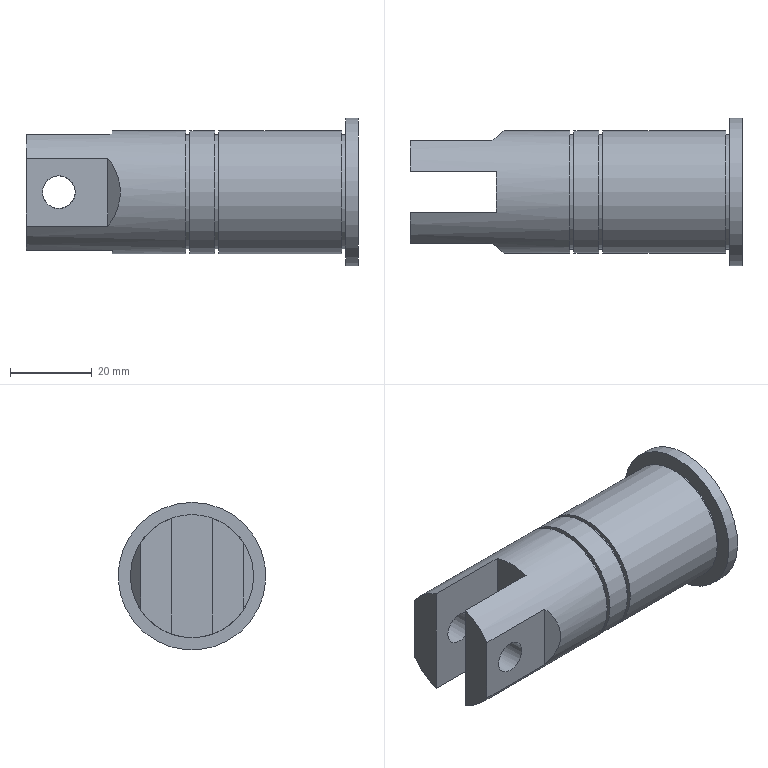Component | NX | PLUNGER | 1 solid | 29 faces | volume 40051 mm3 | plane 17 | cylinder 11 | cone 1 | commonest cylinder face diameters 30 x3 28 x3 8 x2 36 x1 22 x1 10 x1